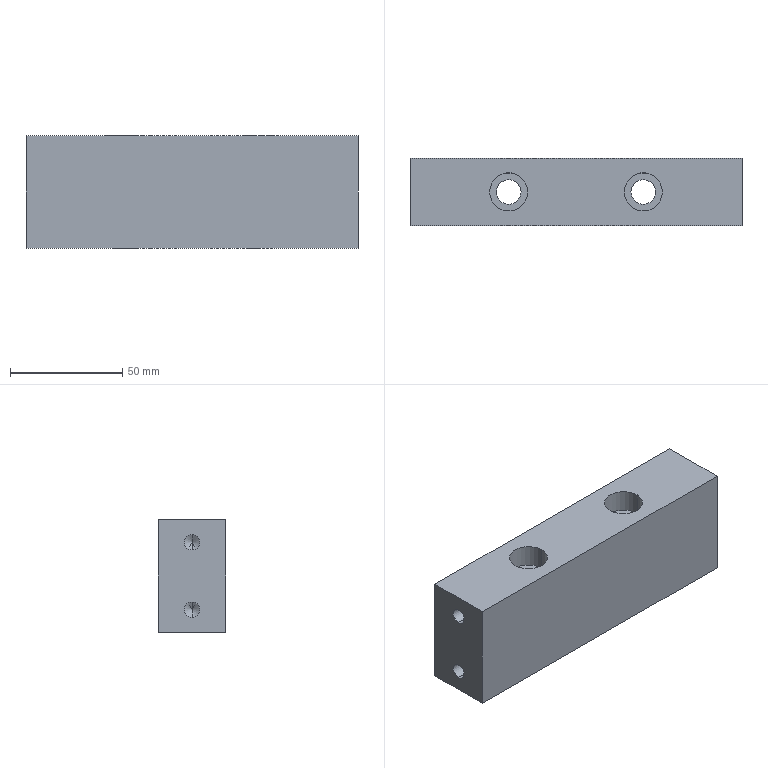Component | SolidWorks | GuideMechanism-1_GuideSeatFixingPlate-1 | 1 solid | 32 faces | box 148 x 30 x 50 mm | volume 207289 mm3 | cylinder 16 | cone 8 | plane 8 | commonest cylinder face diameters 6.8 x8 17 x4 11 x4
build123d program:
from build123d import *

# Parameters (mm, degrees)
SKETCH1_W                                        = 148
SKETCH1_H                                        = 30
BOSS_EXTRUDE1_DEPTH                              = 50
HOLE_SIZE_ACCORDING_TO_TYPE_1_OF_HEX_D           = 11
HOLE_SIZE_ACCORDING_TO_TYPE_1_OF_HEX_CBORE_D     = 17
HOLE_SIZE_ACCORDING_TO_TYPE_1_OF_HEX_CBORE_DEPTH = 10
M8_TAPPED_HOLE1_AT_2_COUNT                       = 2
M8_TAPPED_HOLE1_AT_2_PITCH                       = 30


with BuildPart() as part:
    # Sketch1 → Boss-Extrude1 (new body)
    with BuildSketch(Plane.XY):
        Rectangle(SKETCH1_W, SKETCH1_H)
    extrude(amount=BOSS_EXTRUDE1_DEPTH)

    # Hole Size _ according to_ Type 1 of Hex (through all)
    with Locations(Plane.XY.offset(50)):
        with Locations((-30, 0), (30, 0)):
            CounterBoreHole(HOLE_SIZE_ACCORDING_TO_TYPE_1_OF_HEX_D / 2, HOLE_SIZE_ACCORDING_TO_TYPE_1_OF_HEX_CBORE_D / 2, HOLE_SIZE_ACCORDING_TO_TYPE_1_OF_HEX_CBORE_DEPTH)

    # Sketch6 → M8 Tapped Hole1 (revolve, cut)
    with BuildSketch(Plane(origin=(74, 0, 40), x_dir=(0, 0, -1), z_dir=(0, 1, 0))):
        Polygon((0, 0), (0, 19.043), (3.4, 17), (3.4, 0), align=None)
    m8_tapped_hole1 = revolve(axis=Axis((80.35, 0, 40), (-1, 0, 0)), mode=Mode.SUBTRACT)

    # M8 Tapped Hole1 at 2: M8 Tapped Hole1 ×2
    with Locations(*[(0, 0, -i * M8_TAPPED_HOLE1_AT_2_PITCH) for i in range(1, M8_TAPPED_HOLE1_AT_2_COUNT)]):
        add(m8_tapped_hole1, mode=Mode.SUBTRACT)

    # Mirror1: M8 Tapped Hole1 across plane
    add(m8_tapped_hole1.mirror(Plane(origin=(0, 0, 0), x_dir=(0, 0, 1), z_dir=(1, 0, 0))), mode=Mode.SUBTRACT)

    # Mirror1 copy 1 sketch → Mirror1 copy 1 (revolve, cut)
    with BuildSketch(Plane(origin=(-74, 0, 10), x_dir=(0, 0, -1), z_dir=(0, 1, 0))):
        Polygon((0, 0), (0, -19.043), (3.4, -17), (3.4, 0), align=None)
    revolve(axis=Axis((-80.35, 0, 10), (-1, 0, 0)), mode=Mode.SUBTRACT)


solid = part.part

# Placed as in the assembly
solid = solid.moved(Location((-439.272, -538.766, 1161.5), (0, 0, 0)))
STEP:
#1=CARTESIAN_POINT('',(-19.538,-21.211,47.169));
#2=VERTEX_POINT('',#1);
#3=CARTESIAN_POINT('',(-19.538,-21.211,47.437));
#4=VERTEX_POINT('',#3);
#5=CARTESIAN_POINT('',(-19.538,-21.211,47.303));
#6=DIRECTION('',(-1.,0.,0.));
#7=DIRECTION('',(0.,0.,1.));
#8=AXIS2_PLACEMENT_3D('',#5,#6,#7);
#9=CIRCLE('',#8,0.1339);
#10=EDGE_CURVE('',#2,#4,#9,.T.);
#11=ORIENTED_EDGE('',*,*,#10,.F.);
#12=CARTESIAN_POINT('',(-20.208,-21.211,47.169));
#13=VERTEX_POINT('',#12);
#14=CARTESIAN_POINT('',(-20.208,-21.211,47.169));
#15=DIRECTION('',(-1.,0.,0.));
#16=VECTOR('',#15,39.37);
#17=LINE('',#14,#16);
#18=EDGE_CURVE('',#2,#13,#17,.T.);
#19=ORIENTED_EDGE('',*,*,#18,.T.);
#20=CARTESIAN_POINT('',(-20.208,-21.211,47.437));
#21=VERTEX_POINT('',#20);
#22=CARTESIAN_POINT('',(-20.208,-21.211,47.303));
#23=DIRECTION('',(-1.,0.,0.));
#24=DIRECTION('',(0.,0.,1.));
#25=AXIS2_PLACEMENT_3D('',#22,#23,#24);
#26=CIRCLE('',#25,0.1339);
#27=EDGE_CURVE('',#13,#21,#26,.T.);
#28=ORIENTED_EDGE('',*,*,#27,.T.);
#29=CARTESIAN_POINT('',(-20.208,-21.211,47.437));
#30=DIRECTION('',(-1.,0.,0.));
#31=VECTOR('',#30,39.37);
#32=LINE('',#29,#31);
#33=EDGE_CURVE('',#4,#21,#32,.T.);
#34=ORIENTED_EDGE('',*,*,#33,.F.);
#35=EDGE_LOOP('',(#11,#19,#28,#34));
#36=FACE_OUTER_BOUND('',#35,.T.);
#37=CARTESIAN_POINT('',(-20.208,-21.211,47.303));
#38=DIRECTION('',(-1.,0.,0.));
#39=DIRECTION('',(0.,0.,1.));
#40=AXIS2_PLACEMENT_3D('',#37,#38,#39);
#41=CYLINDRICAL_SURFACE('',#40,0.1339);
#42=ADVANCED_FACE('',(#36),#41,.F.);
#43=CARTESIAN_POINT('',(-19.458,-21.211,47.303));
#44=VERTEX_POINT('',#43);
#45=CARTESIAN_POINT('',(-19.538,-21.211,47.437));
#46=DIRECTION('',(-0.515,0.,0.8572));
#47=VECTOR('',#46,39.37);
#48=LINE('',#45,#47);
#49=EDGE_CURVE('',#44,#4,#48,.T.);
#50=ORIENTED_EDGE('',*,*,#49,.F.);
#51=CARTESIAN_POINT('',(-19.538,-21.211,47.169));
#52=DIRECTION('',(-0.515,0.,-0.8572));
#53=VECTOR('',#52,39.37);
#54=LINE('',#51,#53);
#55=EDGE_CURVE('',#44,#2,#54,.T.);
#56=ORIENTED_EDGE('',*,*,#55,.T.);
#57=ORIENTED_EDGE('',*,*,#10,.T.);
#58=EDGE_LOOP('',(#50,#56,#57));
#59=FACE_OUTER_BOUND('',#58,.T.);
#60=CARTESIAN_POINT('',(-19.538,-21.211,47.303));
#61=DIRECTION('',(-1.,0.,0.));
#62=DIRECTION('',(0.,0.,1.));
#63=AXIS2_PLACEMENT_3D('',#60,#61,#62);
#64=CONICAL_SURFACE('',#63,0.1339,1.03);
#65=ADVANCED_FACE('',(#59),#64,.F.);
#66=CARTESIAN_POINT('',(-19.538,-21.211,45.988));
#67=VERTEX_POINT('',#66);
#68=CARTESIAN_POINT('',(-19.538,-21.211,46.256));
#69=VERTEX_POINT('',#68);
#70=CARTESIAN_POINT('',(-19.538,-21.211,46.122));
#71=DIRECTION('',(-1.,0.,0.));
#72=DIRECTION('',(0.,0.,1.));
#73=AXIS2_PLACEMENT_3D('',#70,#71,#72);
#74=CIRCLE('',#73,0.1339);
#75=EDGE_CURVE('',#67,#69,#74,.T.);
#76=ORIENTED_EDGE('',*,*,#75,.F.);
#77=CARTESIAN_POINT('',(-20.208,-21.211,45.988));
#78=VERTEX_POINT('',#77);
#79=CARTESIAN_POINT('',(-20.208,-21.211,45.988));
#80=DIRECTION('',(-1.,0.,0.));
#81=VECTOR('',#80,39.37);
#82=LINE('',#79,#81);
#83=EDGE_CURVE('',#67,#78,#82,.T.);
#84=ORIENTED_EDGE('',*,*,#83,.T.);
#85=CARTESIAN_POINT('',(-20.208,-21.211,46.256));
#86=VERTEX_POINT('',#85);
#87=CARTESIAN_POINT('',(-20.208,-21.211,46.122));
#88=DIRECTION('',(-1.,0.,0.));
#89=DIRECTION('',(0.,0.,1.));
#90=AXIS2_PLACEMENT_3D('',#87,#88,#89);
#91=CIRCLE('',#90,0.1339);
#92=EDGE_CURVE('',#78,#86,#91,.T.);
#93=ORIENTED_EDGE('',*,*,#92,.T.);
#94=CARTESIAN_POINT('',(-20.208,-21.211,46.256));
#95=DIRECTION('',(-1.,0.,0.));
#96=VECTOR('',#95,39.37);
#97=LINE('',#94,#96);
#98=EDGE_CURVE('',#69,#86,#97,.T.);
#99=ORIENTED_EDGE('',*,*,#98,.F.);
#100=EDGE_LOOP('',(#76,#84,#93,#99));
#101=FACE_OUTER_BOUND('',#100,.T.);
#102=CARTESIAN_POINT('',(-20.208,-21.211,46.122));
#103=DIRECTION('',(-1.,0.,0.));
#104=DIRECTION('',(0.,0.,1.));
#105=AXIS2_PLACEMENT_3D('',#102,#103,#104);
#106=CYLINDRICAL_SURFACE('',#105,0.1339);
#107=ADVANCED_FACE('',(#101),#106,.F.);
#108=CARTESIAN_POINT('',(-19.458,-21.211,46.122));
#109=VERTEX_POINT('',#108);
#110=CARTESIAN_POINT('',(-19.538,-21.211,46.256));
#111=DIRECTION('',(-0.515,0.,0.8572));
#112=VECTOR('',#111,39.37);
#113=LINE('',#110,#112);
#114=EDGE_CURVE('',#109,#69,#113,.T.);
#115=ORIENTED_EDGE('',*,*,#114,.F.);
#116=CARTESIAN_POINT('',(-19.538,-21.211,45.988));
#117=DIRECTION('',(-0.515,0.,-0.8572));
#118=VECTOR('',#117,39.37);
#119=LINE('',#116,#118);
#120=EDGE_CURVE('',#109,#67,#119,.T.);
#121=ORIENTED_EDGE('',*,*,#120,.T.);
#122=ORIENTED_EDGE('',*,*,#75,.T.);
#123=EDGE_LOOP('',(#115,#121,#122));
#124=FACE_OUTER_BOUND('',#123,.T.);
#125=CARTESIAN_POINT('',(-19.538,-21.211,46.122));
#126=DIRECTION('',(-1.,0.,0.));
#127=DIRECTION('',(0.,0.,1.));
#128=AXIS2_PLACEMENT_3D('',#125,#126,#127);
#129=CONICAL_SURFACE('',#128,0.1339,1.03);
#130=ADVANCED_FACE('',(#124),#129,.F.);
#131=CARTESIAN_POINT('',(-15.05,-21.211,47.437));
#132=VERTEX_POINT('',#131);
#133=CARTESIAN_POINT('',(-15.05,-21.211,47.169));
#134=VERTEX_POINT('',#133);
#135=CARTESIAN_POINT('',(-15.05,-21.211,47.303));
#136=DIRECTION('',(1.,0.,0.));
#137=DIRECTION('',(0.,0.,-1.));
#138=AXIS2_PLACEMENT_3D('',#135,#136,#137);
#139=CIRCLE('',#138,0.1339);
#140=EDGE_CURVE('',#132,#134,#139,.T.);
#141=ORIENTED_EDGE('',*,*,#140,.F.);
#142=CARTESIAN_POINT('',(-14.381,-21.211,47.437));
#143=VERTEX_POINT('',#142);
#144=CARTESIAN_POINT('',(-14.381,-21.211,47.437));
#145=DIRECTION('',(1.,0.,0.));
#146=VECTOR('',#145,39.37);
#147=LINE('',#144,#146);
#148=EDGE_CURVE('',#132,#143,#147,.T.);
#149=ORIENTED_EDGE('',*,*,#148,.T.);
#150=CARTESIAN_POINT('',(-14.381,-21.211,47.169));
#151=VERTEX_POINT('',#150);
#152=CARTESIAN_POINT('',(-14.381,-21.211,47.303));
#153=DIRECTION('',(1.,0.,0.));
#154=DIRECTION('',(0.,0.,-1.));
#155=AXIS2_PLACEMENT_3D('',#152,#153,#154);
#156=CIRCLE('',#155,0.1339);
#157=EDGE_CURVE('',#143,#151,#156,.T.);
#158=ORIENTED_EDGE('',*,*,#157,.T.);
#159=CARTESIAN_POINT('',(-14.381,-21.211,47.169));
#160=DIRECTION('',(1.,0.,0.));
#161=VECTOR('',#160,39.37);
#162=LINE('',#159,#161);
#163=EDGE_CURVE('',#134,#151,#162,.T.);
#164=ORIENTED_EDGE('',*,*,#163,.F.);
#165=EDGE_LOOP('',(#141,#149,#158,#164));
#166=FACE_OUTER_BOUND('',#165,.T.);
#167=CARTESIAN_POINT('',(-14.381,-21.211,47.303));
#168=DIRECTION('',(1.,0.,0.));
#169=DIRECTION('',(0.,0.,-1.));
#170=AXIS2_PLACEMENT_3D('',#167,#168,#169);
#171=CYLINDRICAL_SURFACE('',#170,0.1339);
#172=ADVANCED_FACE('',(#166),#171,.F.);
#173=CARTESIAN_POINT('',(-15.131,-21.211,47.303));
#174=VERTEX_POINT('',#173);
#175=CARTESIAN_POINT('',(-15.05,-21.211,47.169));
#176=DIRECTION('',(0.515,0.,-0.8572));
#177=VECTOR('',#176,39.37);
#178=LINE('',#175,#177);
#179=EDGE_CURVE('',#174,#134,#178,.T.);
#180=ORIENTED_EDGE('',*,*,#179,.F.);
#181=CARTESIAN_POINT('',(-15.05,-21.211,47.437));
#182=DIRECTION('',(0.515,0.,0.8572));
#183=VECTOR('',#182,39.37);
#184=LINE('',#181,#183);
#185=EDGE_CURVE('',#174,#132,#184,.T.);
#186=ORIENTED_EDGE('',*,*,#185,.T.);
#187=ORIENTED_EDGE('',*,*,#140,.T.);
#188=EDGE_LOOP('',(#180,#186,#187));
#189=FACE_OUTER_BOUND('',#188,.T.);
#190=CARTESIAN_POINT('',(-15.05,-21.211,47.303));
#191=DIRECTION('',(1.,0.,0.));
#192=DIRECTION('',(0.,0.,-1.));
#193=AXIS2_PLACEMENT_3D('',#190,#191,#192);
#194=CONICAL_SURFACE('',#193,0.1339,1.03);
#195=ADVANCED_FACE('',(#189),#194,.F.);
#196=CARTESIAN_POINT('',(-15.05,-21.211,46.256));
#197=VERTEX_POINT('',#196);
#198=CARTESIAN_POINT('',(-15.05,-21.211,45.988));
#199=VERTEX_POINT('',#198);
#200=CARTESIAN_POINT('',(-15.05,-21.211,46.122));
#201=DIRECTION('',(1.,0.,0.));
#202=DIRECTION('',(0.,0.,-1.));
#203=AXIS2_PLACEMENT_3D('',#200,#201,#202);
#204=CIRCLE('',#203,0.1339);
#205=EDGE_CURVE('',#197,#199,#204,.T.);
#206=ORIENTED_EDGE('',*,*,#205,.F.);
#207=CARTESIAN_POINT('',(-14.381,-21.211,46.256));
#208=VERTEX_POINT('',#207);
#209=CARTESIAN_POINT('',(-14.381,-21.211,46.256));
#210=DIRECTION('',(1.,0.,0.));
#211=VECTOR('',#210,39.37);
#212=LINE('',#209,#211);
#213=EDGE_CURVE('',#197,#208,#212,.T.);
#214=ORIENTED_EDGE('',*,*,#213,.T.);
#215=CARTESIAN_POINT('',(-14.381,-21.211,45.988));
#216=VERTEX_POINT('',#215);
#217=CARTESIAN_POINT('',(-14.381,-21.211,46.122));
#218=DIRECTION('',(1.,0.,0.));
#219=DIRECTION('',(0.,0.,-1.));
#220=AXIS2_PLACEMENT_3D('',#217,#218,#219);
#221=CIRCLE('',#220,0.1339);
#222=EDGE_CURVE('',#208,#216,#221,.T.);
#223=ORIENTED_EDGE('',*,*,#222,.T.);
#224=CARTESIAN_POINT('',(-14.381,-21.211,45.988));
#225=DIRECTION('',(1.,0.,0.));
#226=VECTOR('',#225,39.37);
#227=LINE('',#224,#226);
#228=EDGE_CURVE('',#199,#216,#227,.T.);
#229=ORIENTED_EDGE('',*,*,#228,.F.);
#230=EDGE_LOOP('',(#206,#214,#223,#229));
#231=FACE_OUTER_BOUND('',#230,.T.);
#232=CARTESIAN_POINT('',(-14.381,-21.211,46.122));
#233=DIRECTION('',(1.,0.,0.));
#234=DIRECTION('',(0.,0.,-1.));
#235=AXIS2_PLACEMENT_3D('',#232,#233,#234);
#236=CYLINDRICAL_SURFACE('',#235,0.1339);
#237=ADVANCED_FACE('',(#231),#236,.F.);
#238=CARTESIAN_POINT('',(-15.131,-21.211,46.122));
#239=VERTEX_POINT('',#238);
#240=CARTESIAN_POINT('',(-15.05,-21.211,45.988));
#241=DIRECTION('',(0.515,0.,-0.8572));
#242=VECTOR('',#241,39.37);
#243=LINE('',#240,#242);
#244=EDGE_CURVE('',#239,#199,#243,.T.);
#245=ORIENTED_EDGE('',*,*,#244,.F.);
#246=CARTESIAN_POINT('',(-15.05,-21.211,46.256));
#247=DIRECTION('',(0.515,0.,0.8572));
#248=VECTOR('',#247,39.37);
#249=LINE('',#246,#248);
#250=EDGE_CURVE('',#239,#197,#249,.T.);
#251=ORIENTED_EDGE('',*,*,#250,.T.);
#252=ORIENTED_EDGE('',*,*,#205,.T.);
#253=EDGE_LOOP('',(#245,#251,#252));
#254=FACE_OUTER_BOUND('',#253,.T.);
#255=CARTESIAN_POINT('',(-15.05,-21.211,46.122));
#256=DIRECTION('',(1.,0.,0.));
#257=DIRECTION('',(0.,0.,-1.));
#258=AXIS2_PLACEMENT_3D('',#255,#256,#257);
#259=CONICAL_SURFACE('',#258,0.1339,1.03);
#260=ADVANCED_FACE('',(#254),#259,.F.);
#261=CARTESIAN_POINT('',(-18.81,-21.211,47.303));
#262=VERTEX_POINT('',#261);
#263=CARTESIAN_POINT('',(-18.141,-21.211,47.303));
#264=VERTEX_POINT('',#263);
#265=CARTESIAN_POINT('',(-18.475,-21.211,47.303));
#266=DIRECTION('',(0.,0.,1.));
#267=DIRECTION('',(1.,0.,0.));
#268=AXIS2_PLACEMENT_3D('',#265,#266,#267);
#269=CIRCLE('',#268,0.3346);
#270=EDGE_CURVE('',#262,#264,#269,.T.);
#271=ORIENTED_EDGE('',*,*,#270,.F.);
#272=CARTESIAN_POINT('',(-18.81,-21.211,47.697));
#273=VERTEX_POINT('',#272);
#274=CARTESIAN_POINT('',(-18.81,-21.211,47.697));
#275=DIRECTION('',(0.,0.,1.));
#276=VECTOR('',#275,39.37);
#277=LINE('',#274,#276);
#278=EDGE_CURVE('',#262,#273,#277,.T.);
#279=ORIENTED_EDGE('',*,*,#278,.T.);
#280=CARTESIAN_POINT('',(-18.141,-21.211,47.697));
#281=VERTEX_POINT('',#280);
#282=CARTESIAN_POINT('',(-18.475,-21.211,47.697));
#283=DIRECTION('',(0.,0.,1.));
#284=DIRECTION('',(1.,0.,0.));
#285=AXIS2_PLACEMENT_3D('',#282,#283,#284);
#286=CIRCLE('',#285,0.3346);
#287=EDGE_CURVE('',#273,#281,#286,.T.);
#288=ORIENTED_EDGE('',*,*,#287,.T.);
#289=CARTESIAN_POINT('',(-18.141,-21.211,47.697));
#290=DIRECTION('',(0.,0.,1.));
#291=VECTOR('',#290,39.37);
#292=LINE('',#289,#291);
#293=EDGE_CURVE('',#264,#281,#292,.T.);
#294=ORIENTED_EDGE('',*,*,#293,.F.);
#295=EDGE_LOOP('',(#271,#279,#288,#294));
#296=FACE_OUTER_BOUND('',#295,.T.);
#297=CARTESIAN_POINT('',(-18.475,-21.211,47.697));
#298=DIRECTION('',(0.,0.,1.));
#299=DIRECTION('',(1.,0.,0.));
#300=AXIS2_PLACEMENT_3D('',#297,#298,#299);
#301=CYLINDRICAL_SURFACE('',#300,0.3346);
#302=ADVANCED_FACE('',(#296),#301,.F.);
#303=CARTESIAN_POINT('',(-18.692,-21.211,45.728));
#304=VERTEX_POINT('',#303);
#305=CARTESIAN_POINT('',(-18.259,-21.211,45.728));
#306=VERTEX_POINT('',#305);
#307=CARTESIAN_POINT('',(-18.475,-21.211,45.728));
#308=DIRECTION('',(0.,0.,1.));
#309=DIRECTION('',(1.,0.,0.));
#310=AXIS2_PLACEMENT_3D('',#307,#308,#309);
#311=CIRCLE('',#310,0.2165);
#312=EDGE_CURVE('',#304,#306,#311,.T.);
#313=ORIENTED_EDGE('',*,*,#312,.F.);
#314=CARTESIAN_POINT('',(-18.692,-21.211,47.303));
#315=VERTEX_POINT('',#314);
#316=CARTESIAN_POINT('',(-18.692,-21.211,47.697));
#317=DIRECTION('',(0.,0.,1.));
#318=VECTOR('',#317,39.37);
#319=LINE('',#316,#318);
#320=EDGE_CURVE('',#304,#315,#319,.T.);
#321=ORIENTED_EDGE('',*,*,#320,.T.);
#322=CARTESIAN_POINT('',(-18.259,-21.211,47.303));
#323=VERTEX_POINT('',#322);
#324=CARTESIAN_POINT('',(-18.475,-21.211,47.303));
#325=DIRECTION('',(0.,0.,1.));
#326=DIRECTION('',(1.,0.,0.));
#327=AXIS2_PLACEMENT_3D('',#324,#325,#326);
#328=CIRCLE('',#327,0.2165);
#329=EDGE_CURVE('',#315,#323,#328,.T.);
#330=ORIENTED_EDGE('',*,*,#329,.T.);
#331=CARTESIAN_POINT('',(-18.259,-21.211,47.697));
#332=DIRECTION('',(0.,0.,1.));
#333=VECTOR('',#332,39.37);
#334=LINE('',#331,#333);
#335=EDGE_CURVE('',#306,#323,#334,.T.);
#336=ORIENTED_EDGE('',*,*,#335,.F.);
#337=EDGE_LOOP('',(#313,#321,#330,#336));
#338=FACE_OUTER_BOUND('',#337,.T.);
#339=CARTESIAN_POINT('',(-18.475,-21.211,47.697));
#340=DIRECTION('',(0.,0.,1.));
#341=DIRECTION('',(1.,0.,0.));
#342=AXIS2_PLACEMENT_3D('',#339,#340,#341);
#343=CYLINDRICAL_SURFACE('',#342,0.2165);
#344=ADVANCED_FACE('',(#338),#343,.F.);
#345=CARTESIAN_POINT('',(-16.448,-21.211,47.303));
#346=VERTEX_POINT('',#345);
#347=CARTESIAN_POINT('',(-15.778,-21.211,47.303));
#348=VERTEX_POINT('',#347);
#349=CARTESIAN_POINT('',(-16.113,-21.211,47.303));
#350=DIRECTION('',(0.,0.,1.));
#351=DIRECTION('',(1.,0.,0.));
#352=AXIS2_PLACEMENT_3D('',#349,#350,#351);
#353=CIRCLE('',#352,0.3346);
#354=EDGE_CURVE('',#346,#348,#353,.T.);
#355=ORIENTED_EDGE('',*,*,#354,.F.);
#356=CARTESIAN_POINT('',(-16.448,-21.211,47.697));
#357=VERTEX_POINT('',#356);
#358=CARTESIAN_POINT('',(-16.448,-21.211,47.697));
#359=DIRECTION('',(0.,0.,1.));
#360=VECTOR('',#359,39.37);
#361=LINE('',#358,#360);
#362=EDGE_CURVE('',#346,#357,#361,.T.);
#363=ORIENTED_EDGE('',*,*,#362,.T.);
#364=CARTESIAN_POINT('',(-15.778,-21.211,47.697));
#365=VERTEX_POINT('',#364);
#366=CARTESIAN_POINT('',(-16.113,-21.211,47.697));
#367=DIRECTION('',(0.,0.,1.));
#368=DIRECTION('',(1.,0.,0.));
#369=AXIS2_PLACEMENT_3D('',#366,#367,#368);
#370=CIRCLE('',#369,0.3346);
#371=EDGE_CURVE('',#357,#365,#370,.T.);
#372=ORIENTED_EDGE('',*,*,#371,.T.);
#373=CARTESIAN_POINT('',(-15.778,-21.211,47.697));
#374=DIRECTION('',(0.,0.,1.));
#375=VECTOR('',#374,39.37);
#376=LINE('',#373,#375);
#377=EDGE_CURVE('',#348,#365,#376,.T.);
#378=ORIENTED_EDGE('',*,*,#377,.F.);
#379=EDGE_LOOP('',(#355,#363,#372,#378));
#380=FACE_OUTER_BOUND('',#379,.T.);
#381=CARTESIAN_POINT('',(-16.113,-21.211,47.697));
#382=DIRECTION('',(0.,0.,1.));
#383=DIRECTION('',(1.,0.,0.));
#384=AXIS2_PLACEMENT_3D('',#381,#382,#383);
#385=CYLINDRICAL_SURFACE('',#384,0.3346);
#386=ADVANCED_FACE('',(#380),#385,.F.);
#387=CARTESIAN_POINT('',(-16.33,-21.211,45.728));
#388=VERTEX_POINT('',#387);
#389=CARTESIAN_POINT('',(-15.897,-21.211,45.728));
#390=VERTEX_POINT('',#389);
#391=CARTESIAN_POINT('',(-16.113,-21.211,45.728));
#392=DIRECTION('',(0.,0.,1.));
#393=DIRECTION('',(1.,0.,0.));
#394=AXIS2_PLACEMENT_3D('',#391,#392,#393);
#395=CIRCLE('',#394,0.2165);
#396=EDGE_CURVE('',#388,#390,#395,.T.);
#397=ORIENTED_EDGE('',*,*,#396,.F.);
#398=CARTESIAN_POINT('',(-16.33,-21.211,47.303));
#399=VERTEX_POINT('',#398);
#400=CARTESIAN_POINT('',(-16.33,-21.211,47.697));
#401=DIRECTION('',(0.,0.,1.));
#402=VECTOR('',#401,39.37);
#403=LINE('',#400,#402);
#404=EDGE_CURVE('',#388,#399,#403,.T.);
#405=ORIENTED_EDGE('',*,*,#404,.T.);
#406=CARTESIAN_POINT('',(-15.897,-21.211,47.303));
#407=VERTEX_POINT('',#406);
#408=CARTESIAN_POINT('',(-16.113,-21.211,47.303));
#409=DIRECTION('',(0.,0.,1.));
#410=DIRECTION('',(1.,0.,0.));
#411=AXIS2_PLACEMENT_3D('',#408,#409,#410);
#412=CIRCLE('',#411,0.2165);
#413=EDGE_CURVE('',#399,#407,#412,.T.);
#414=ORIENTED_EDGE('',*,*,#413,.T.);
#415=CARTESIAN_POINT('',(-15.897,-21.211,47.697));
#416=DIRECTION('',(0.,0.,1.));
#417=VECTOR('',#416,39.37);
#418=LINE('',#415,#417);
#419=EDGE_CURVE('',#390,#407,#418,.T.);
#420=ORIENTED_EDGE('',*,*,#419,.F.);
#421=EDGE_LOOP('',(#397,#405,#414,#420));
#422=FACE_OUTER_BOUND('',#421,.T.);
#423=CARTESIAN_POINT('',(-16.113,-21.211,47.697));
#424=DIRECTION('',(0.,0.,1.));
#425=DIRECTION('',(1.,0.,0.));
#426=AXIS2_PLACEMENT_3D('',#423,#424,#425);
#427=CYLINDRICAL_SURFACE('',#426,0.2165);
#428=ADVANCED_FACE('',(#422),#427,.F.);
#429=CARTESIAN_POINT('',(-20.208,-21.211,47.303));
#430=DIRECTION('',(-1.,0.,0.));
#431=DIRECTION('',(0.,0.,1.));
#432=AXIS2_PLACEMENT_3D('',#429,#430,#431);
#433=CIRCLE('',#432,0.1339);
#434=EDGE_CURVE('',#21,#13,#433,.T.);
#435=ORIENTED_EDGE('',*,*,#434,.F.);
#436=ORIENTED_EDGE('',*,*,#27,.F.);
#437=EDGE_LOOP('',(#435,#436));
#438=FACE_BOUND('',#437,.T.);
#439=CARTESIAN_POINT('',(-20.208,-21.211,46.122));
#440=DIRECTION('',(-1.,0.,0.));
#441=DIRECTION('',(0.,0.,1.));
#442=AXIS2_PLACEMENT_3D('',#439,#440,#441);
#443=CIRCLE('',#442,0.1339);
#444=EDGE_CURVE('',#86,#78,#443,.T.);
#445=ORIENTED_EDGE('',*,*,#444,.F.);
#446=ORIENTED_EDGE('',*,*,#92,.F.);
#447=EDGE_LOOP('',(#445,#446));
#448=FACE_BOUND('',#447,.T.);
#449=CARTESIAN_POINT('',(-20.208,-20.621,45.728));
#450=VERTEX_POINT('',#449);
#451=CARTESIAN_POINT('',(-20.208,-21.802,45.728));
#452=VERTEX_POINT('',#451);
#453=CARTESIAN_POINT('',(-20.208,-21.802,45.728));
#454=DIRECTION('',(0.,-1.,0.));
#455=VECTOR('',#454,39.37);
#456=LINE('',#453,#455);
#457=EDGE_CURVE('',#450,#452,#456,.T.);
#458=ORIENTED_EDGE('',*,*,#457,.T.);
#459=CARTESIAN_POINT('',(-20.208,-21.802,47.697));
#460=VERTEX_POINT('',#459);
#461=CARTESIAN_POINT('',(-20.208,-21.802,47.697));
#462=DIRECTION('',(0.,0.,-1.));
#463=VECTOR('',#462,39.37);
#464=LINE('',#461,#463);
#465=EDGE_CURVE('',#460,#452,#464,.T.);
#466=ORIENTED_EDGE('',*,*,#465,.F.);
#467=CARTESIAN_POINT('',(-20.208,-20.621,47.697));
#468=VERTEX_POINT('',#467);
#469=CARTESIAN_POINT('',(-20.208,-21.802,47.697));
#470=DIRECTION('',(0.,-1.,0.));
#471=VECTOR('',#470,39.37);
#472=LINE('',#469,#471);
#473=EDGE_CURVE('',#468,#460,#472,.T.);
#474=ORIENTED_EDGE('',*,*,#473,.F.);
#475=CARTESIAN_POINT('',(-20.208,-20.621,47.697));
#476=DIRECTION('',(0.,0.,-1.));
#477=VECTOR('',#476,39.37);
#478=LINE('',#475,#477);
#479=EDGE_CURVE('',#468,#450,#478,.T.);
#480=ORIENTED_EDGE('',*,*,#479,.T.);
#481=EDGE_LOOP('',(#458,#466,#474,#480));
#482=FACE_OUTER_BOUND('',#481,.T.);
#483=CARTESIAN_POINT('',(-20.208,-21.802,47.697));
#484=DIRECTION('',(1.,0.,0.));
#485=DIRECTION('',(0.,0.,-1.));
#486=AXIS2_PLACEMENT_3D('',#483,#484,#485);
#487=PLANE('',#486);
#488=ADVANCED_FACE('',(#438,#448,#482),#487,.F.);
#489=CARTESIAN_POINT('',(-14.381,-21.802,45.728));
#490=VERTEX_POINT('',#489);
#491=CARTESIAN_POINT('',(-14.381,-21.802,45.728));
#492=DIRECTION('',(1.,0.,0.));
#493=VECTOR('',#492,39.37);
#494=LINE('',#491,#493);
#495=EDGE_CURVE('',#452,#490,#494,.T.);
#496=ORIENTED_EDGE('',*,*,#495,.T.);
#497=CARTESIAN_POINT('',(-14.381,-21.802,47.697));
#498=VERTEX_POINT('',#497);
#499=CARTESIAN_POINT('',(-14.381,-21.802,47.697));
#500=DIRECTION('',(0.,0.,-1.));
#501=VECTOR('',#500,39.37);
#502=LINE('',#499,#501);
#503=EDGE_CURVE('',#498,#490,#502,.T.);
#504=ORIENTED_EDGE('',*,*,#503,.F.);
#505=CARTESIAN_POINT('',(-14.381,-21.802,47.697));
#506=DIRECTION('',(1.,0.,0.));
#507=VECTOR('',#506,39.37);
#508=LINE('',#505,#507);
#509=EDGE_CURVE('',#460,#498,#508,.T.);
#510=ORIENTED_EDGE('',*,*,#509,.F.);
#511=ORIENTED_EDGE('',*,*,#465,.T.);
#512=EDGE_LOOP('',(#496,#504,#510,#511));
#513=FACE_OUTER_BOUND('',#512,.T.);
#514=CARTESIAN_POINT('',(-14.381,-21.802,47.697));
#515=DIRECTION('',(-0.,1.,0.));
#516=DIRECTION('',(-1.,-0.,0.));
#517=AXIS2_PLACEMENT_3D('',#514,#515,#516);
#518=PLANE('',#517);
#519=ADVANCED_FACE('',(#513),#518,.F.);
#520=CARTESIAN_POINT('',(-14.381,-21.211,47.303));
#521=DIRECTION('',(1.,0.,0.));
#522=DIRECTION('',(0.,0.,-1.));
#523=AXIS2_PLACEMENT_3D('',#520,#521,#522);
#524=CIRCLE('',#523,0.1339);
#525=EDGE_CURVE('',#151,#143,#524,.T.);
#526=ORIENTED_EDGE('',*,*,#525,.F.);
#527=ORIENTED_EDGE('',*,*,#157,.F.);
#528=EDGE_LOOP('',(#526,#527));
#529=FACE_BOUND('',#528,.T.);
#530=CARTESIAN_POINT('',(-14.381,-21.211,46.122));
#531=DIRECTION('',(1.,0.,0.));
#532=DIRECTION('',(0.,0.,-1.));
#533=AXIS2_PLACEMENT_3D('',#530,#531,#532);
#534=CIRCLE('',#533,0.1339);
#535=EDGE_CURVE('',#216,#208,#534,.T.);
#536=ORIENTED_EDGE('',*,*,#535,.F.);
#537=ORIENTED_EDGE('',*,*,#222,.F.);
#538=EDGE_LOOP('',(#536,#537));
#539=FACE_BOUND('',#538,.T.);
#540=CARTESIAN_POINT('',(-14.381,-20.621,45.728));
#541=VERTEX_POINT('',#540);
#542=CARTESIAN_POINT('',(-14.381,-21.802,45.728));
#543=DIRECTION('',(0.,1.,0.));
#544=VECTOR('',#543,39.37);
#545=LINE('',#542,#544);
#546=EDGE_CURVE('',#490,#541,#545,.T.);
#547=ORIENTED_EDGE('',*,*,#546,.T.);
#548=CARTESIAN_POINT('',(-14.381,-20.621,47.697));
#549=VERTEX_POINT('',#548);
#550=CARTESIAN_POINT('',(-14.381,-20.621,47.697));
#551=DIRECTION('',(0.,0.,-1.));
#552=VECTOR('',#551,39.37);
#553=LINE('',#550,#552);
#554=EDGE_CURVE('',#549,#541,#553,.T.);
#555=ORIENTED_EDGE('',*,*,#554,.F.);
#556=CARTESIAN_POINT('',(-14.381,-21.802,47.697));
#557=DIRECTION('',(0.,1.,0.));
#558=VECTOR('',#557,39.37);
#559=LINE('',#556,#558);
#560=EDGE_CURVE('',#498,#549,#559,.T.);
#561=ORIENTED_EDGE('',*,*,#560,.F.);
#562=ORIENTED_EDGE('',*,*,#503,.T.);
#563=EDGE_LOOP('',(#547,#555,#561,#562));
#564=FACE_OUTER_BOUND('',#563,.T.);
#565=CARTESIAN_POINT('',(-14.381,-21.802,47.697));
#566=DIRECTION('',(-1.,0.,0.));
#567=DIRECTION('',(0.,0.,1.));
#568=AXIS2_PLACEMENT_3D('',#565,#566,#567);
#569=PLANE('',#568);
#570=ADVANCED_FACE('',(#529,#539,#564),#569,.F.);
#571=CARTESIAN_POINT('',(-14.381,-20.621,45.728));
#572=DIRECTION('',(-1.,-0.,0.));
#573=VECTOR('',#572,39.37);
#574=LINE('',#571,#573);
#575=EDGE_CURVE('',#541,#450,#574,.T.);
#576=ORIENTED_EDGE('',*,*,#575,.T.);
#577=ORIENTED_EDGE('',*,*,#479,.F.);
#578=CARTESIAN_POINT('',(-14.381,-20.621,47.697));
#579=DIRECTION('',(-1.,-0.,0.));
#580=VECTOR('',#579,39.37);
#581=LINE('',#578,#580);
#582=EDGE_CURVE('',#549,#468,#581,.T.);
#583=ORIENTED_EDGE('',*,*,#582,.F.);
#584=ORIENTED_EDGE('',*,*,#554,.T.);
#585=EDGE_LOOP('',(#576,#577,#583,#584));
#586=FACE_OUTER_BOUND('',#585,.T.);
#587=CARTESIAN_POINT('',(-14.381,-20.621,47.697));
#588=DIRECTION('',(0.,-1.,0.));
#589=DIRECTION('',(1.,0.,0.));
#590=AXIS2_PLACEMENT_3D('',#587,#588,#589);
#591=PLANE('',#590);
#592=ADVANCED_FACE('',(#586),#591,.F.);
#593=CARTESIAN_POINT('',(-18.475,-21.211,47.697));
#594=DIRECTION('',(0.,0.,1.));
#595=DIRECTION('',(1.,0.,0.));
#596=AXIS2_PLACEMENT_3D('',#593,#594,#595);
#597=CIRCLE('',#596,0.3346);
#598=EDGE_CURVE('',#281,#273,#597,.T.);
#599=ORIENTED_EDGE('',*,*,#598,.F.);
#600=ORIENTED_EDGE('',*,*,#287,.F.);
#601=EDGE_LOOP('',(#599,#600));
#602=FACE_BOUND('',#601,.T.);
#603=CARTESIAN_POINT('',(-16.113,-21.211,47.697));
#604=DIRECTION('',(0.,0.,1.));
#605=DIRECTION('',(1.,0.,0.));
#606=AXIS2_PLACEMENT_3D('',#603,#604,#605);
#607=CIRCLE('',#606,0.3346);
#608=EDGE_CURVE('',#365,#357,#607,.T.);
#609=ORIENTED_EDGE('',*,*,#608,.F.);
#610=ORIENTED_EDGE('',*,*,#371,.F.);
#611=EDGE_LOOP('',(#609,#610));
#612=FACE_BOUND('',#611,.T.);
#613=ORIENTED_EDGE('',*,*,#473,.T.);
#614=ORIENTED_EDGE('',*,*,#509,.T.);
#615=ORIENTED_EDGE('',*,*,#560,.T.);
#616=ORIENTED_EDGE('',*,*,#582,.T.);
#617=EDGE_LOOP('',(#613,#614,#615,#616));
#618=FACE_OUTER_BOUND('',#617,.T.);
#619=CARTESIAN_POINT('',(-17.294,-21.211,47.697));
#620=DIRECTION('',(0.,0.,1.));
#621=DIRECTION('',(1.,0.,0.));
#622=AXIS2_PLACEMENT_3D('',#619,#620,#621);
#623=PLANE('',#622);
#624=ADVANCED_FACE('',(#602,#612,#618),#623,.T.);
#625=CARTESIAN_POINT('',(-18.475,-21.211,45.728));
#626=DIRECTION('',(0.,0.,1.));
#627=DIRECTION('',(1.,0.,0.));
#628=AXIS2_PLACEMENT_3D('',#625,#626,#627);
#629=CIRCLE('',#628,0.2165);
#630=EDGE_CURVE('',#306,#304,#629,.T.);
#631=ORIENTED_EDGE('',*,*,#630,.T.);
#632=ORIENTED_EDGE('',*,*,#312,.T.);
#633=EDGE_LOOP('',(#631,#632));
#634=FACE_BOUND('',#633,.T.);
#635=CARTESIAN_POINT('',(-16.113,-21.211,45.728));
#636=DIRECTION('',(0.,0.,1.));
#637=DIRECTION('',(1.,0.,0.));
#638=AXIS2_PLACEMENT_3D('',#635,#636,#637);
#639=CIRCLE('',#638,0.2165);
#640=EDGE_CURVE('',#390,#388,#639,.T.);
#641=ORIENTED_EDGE('',*,*,#640,.T.);
#642=ORIENTED_EDGE('',*,*,#396,.T.);
#643=EDGE_LOOP('',(#641,#642));
#644=FACE_BOUND('',#643,.T.);
#645=ORIENTED_EDGE('',*,*,#457,.F.);
#646=ORIENTED_EDGE('',*,*,#575,.F.);
#647=ORIENTED_EDGE('',*,*,#546,.F.);
#648=ORIENTED_EDGE('',*,*,#495,.F.);
#649=EDGE_LOOP('',(#645,#646,#647,#648));
#650=FACE_OUTER_BOUND('',#649,.T.);
#651=CARTESIAN_POINT('',(-17.294,-21.211,45.728));
#652=DIRECTION('',(0.,0.,1.));
#653=DIRECTION('',(1.,0.,0.));
#654=AXIS2_PLACEMENT_3D('',#651,#652,#653);
#655=PLANE('',#654);
#656=ADVANCED_FACE('',(#634,#644,#650),#655,.F.);
#657=ORIENTED_EDGE('',*,*,#404,.F.);
#658=ORIENTED_EDGE('',*,*,#640,.F.);
#659=ORIENTED_EDGE('',*,*,#419,.T.);
#660=CARTESIAN_POINT('',(-16.113,-21.211,47.303));
#661=DIRECTION('',(0.,0.,1.));
#662=DIRECTION('',(1.,0.,0.));
#663=AXIS2_PLACEMENT_3D('',#660,#661,#662);
#664=CIRCLE('',#663,0.2165);
#665=EDGE_CURVE('',#407,#399,#664,.T.);
#666=ORIENTED_EDGE('',*,*,#665,.T.);
#667=EDGE_LOOP('',(#657,#658,#659,#666));
#668=FACE_OUTER_BOUND('',#667,.T.);
#669=CARTESIAN_POINT('',(-16.113,-21.211,47.697));
#670=DIRECTION('',(0.,0.,1.));
#671=DIRECTION('',(1.,0.,0.));
#672=AXIS2_PLACEMENT_3D('',#669,#670,#671);
#673=CYLINDRICAL_SURFACE('',#672,0.2165);
#674=ADVANCED_FACE('',(#668),#673,.F.);
#675=ORIENTED_EDGE('',*,*,#665,.F.);
#676=ORIENTED_EDGE('',*,*,#413,.F.);
#677=EDGE_LOOP('',(#675,#676));
#678=FACE_BOUND('',#677,.T.);
#679=CARTESIAN_POINT('',(-16.113,-21.211,47.303));
#680=DIRECTION('',(0.,0.,1.));
#681=DIRECTION('',(1.,0.,0.));
#682=AXIS2_PLACEMENT_3D('',#679,#680,#681);
#683=CIRCLE('',#682,0.3346);
#684=EDGE_CURVE('',#348,#346,#683,.T.);
#685=ORIENTED_EDGE('',*,*,#684,.T.);
#686=ORIENTED_EDGE('',*,*,#354,.T.);
#687=EDGE_LOOP('',(#685,#686));
#688=FACE_OUTER_BOUND('',#687,.T.);
#689=CARTESIAN_POINT('',(-15.897,-21.211,47.303));
#690=DIRECTION('',(0.,0.,-1.));
#691=DIRECTION('',(-1.,0.,0.));
#692=AXIS2_PLACEMENT_3D('',#689,#690,#691);
#693=PLANE('',#692);
#694=ADVANCED_FACE('',(#678,#688),#693,.F.);
#695=ORIENTED_EDGE('',*,*,#362,.F.);
#696=ORIENTED_EDGE('',*,*,#684,.F.);
#697=ORIENTED_EDGE('',*,*,#377,.T.);
#698=ORIENTED_EDGE('',*,*,#608,.T.);
#699=EDGE_LOOP('',(#695,#696,#697,#698));
#700=FACE_OUTER_BOUND('',#699,.T.);
#701=CARTESIAN_POINT('',(-16.113,-21.211,47.697));
#702=DIRECTION('',(0.,0.,1.));
#703=DIRECTION('',(1.,0.,0.));
#704=AXIS2_PLACEMENT_3D('',#701,#702,#703);
#705=CYLINDRICAL_SURFACE('',#704,0.3346);
#706=ADVANCED_FACE('',(#700),#705,.F.);
#707=ORIENTED_EDGE('',*,*,#320,.F.);
#708=ORIENTED_EDGE('',*,*,#630,.F.);
#709=ORIENTED_EDGE('',*,*,#335,.T.);
#710=CARTESIAN_POINT('',(-18.475,-21.211,47.303));
#711=DIRECTION('',(0.,0.,1.));
#712=DIRECTION('',(1.,0.,0.));
#713=AXIS2_PLACEMENT_3D('',#710,#711,#712);
#714=CIRCLE('',#713,0.2165);
#715=EDGE_CURVE('',#323,#315,#714,.T.);
#716=ORIENTED_EDGE('',*,*,#715,.T.);
#717=EDGE_LOOP('',(#707,#708,#709,#716));
#718=FACE_OUTER_BOUND('',#717,.T.);
#719=CARTESIAN_POINT('',(-18.475,-21.211,47.697));
#720=DIRECTION('',(0.,0.,1.));
#721=DIRECTION('',(1.,0.,0.));
#722=AXIS2_PLACEMENT_3D('',#719,#720,#721);
#723=CYLINDRICAL_SURFACE('',#722,0.2165);
#724=ADVANCED_FACE('',(#718),#723,.F.);
#725=ORIENTED_EDGE('',*,*,#715,.F.);
#726=ORIENTED_EDGE('',*,*,#329,.F.);
#727=EDGE_LOOP('',(#725,#726));
#728=FACE_BOUND('',#727,.T.);
#729=CARTESIAN_POINT('',(-18.475,-21.211,47.303));
#730=DIRECTION('',(0.,0.,1.));
#731=DIRECTION('',(1.,0.,0.));
#732=AXIS2_PLACEMENT_3D('',#729,#730,#731);
#733=CIRCLE('',#732,0.3346);
#734=EDGE_CURVE('',#264,#262,#733,.T.);
#735=ORIENTED_EDGE('',*,*,#734,.T.);
#736=ORIENTED_EDGE('',*,*,#270,.T.);
#737=EDGE_LOOP('',(#735,#736));
#738=FACE_OUTER_BOUND('',#737,.T.);
#739=CARTESIAN_POINT('',(-18.259,-21.211,47.303));
#740=DIRECTION('',(0.,0.,-1.));
#741=DIRECTION('',(-1.,0.,0.));
#742=AXIS2_PLACEMENT_3D('',#739,#740,#741);
#743=PLANE('',#742);
#744=ADVANCED_FACE('',(#728,#738),#743,.F.);
#745=ORIENTED_EDGE('',*,*,#278,.F.);
#746=ORIENTED_EDGE('',*,*,#734,.F.);
#747=ORIENTED_EDGE('',*,*,#293,.T.);
#748=ORIENTED_EDGE('',*,*,#598,.T.);
#749=EDGE_LOOP('',(#745,#746,#747,#748));
#750=FACE_OUTER_BOUND('',#749,.T.);
#751=CARTESIAN_POINT('',(-18.475,-21.211,47.697));
#752=DIRECTION('',(0.,0.,1.));
#753=DIRECTION('',(1.,0.,0.));
#754=AXIS2_PLACEMENT_3D('',#751,#752,#753);
#755=CYLINDRICAL_SURFACE('',#754,0.3346);
#756=ADVANCED_FACE('',(#750),#755,.F.);
#757=ORIENTED_EDGE('',*,*,#250,.F.);
#758=ORIENTED_EDGE('',*,*,#244,.T.);
#759=CARTESIAN_POINT('',(-15.05,-21.211,46.122));
#760=DIRECTION('',(1.,0.,0.));
#761=DIRECTION('',(0.,0.,-1.));
#762=AXIS2_PLACEMENT_3D('',#759,#760,#761);
#763=CIRCLE('',#762,0.1339);
#764=EDGE_CURVE('',#199,#197,#763,.T.);
#765=ORIENTED_EDGE('',*,*,#764,.T.);
#766=EDGE_LOOP('',(#757,#758,#765));
#767=FACE_OUTER_BOUND('',#766,.T.);
#768=CARTESIAN_POINT('',(-15.05,-21.211,46.122));
#769=DIRECTION('',(1.,0.,0.));
#770=DIRECTION('',(0.,0.,-1.));
#771=AXIS2_PLACEMENT_3D('',#768,#769,#770);
#772=CONICAL_SURFACE('',#771,0.1339,1.03);
#773=ADVANCED_FACE('',(#767),#772,.F.);
#774=ORIENTED_EDGE('',*,*,#213,.F.);
#775=ORIENTED_EDGE('',*,*,#764,.F.);
#776=ORIENTED_EDGE('',*,*,#228,.T.);
#777=ORIENTED_EDGE('',*,*,#535,.T.);
#778=EDGE_LOOP('',(#774,#775,#776,#777));
#779=FACE_OUTER_BOUND('',#778,.T.);
#780=CARTESIAN_POINT('',(-14.381,-21.211,46.122));
#781=DIRECTION('',(1.,0.,0.));
#782=DIRECTION('',(0.,0.,-1.));
#783=AXIS2_PLACEMENT_3D('',#780,#781,#782);
#784=CYLINDRICAL_SURFACE('',#783,0.1339);
#785=ADVANCED_FACE('',(#779),#784,.F.);
#786=ORIENTED_EDGE('',*,*,#185,.F.);
#787=ORIENTED_EDGE('',*,*,#179,.T.);
#788=CARTESIAN_POINT('',(-15.05,-21.211,47.303));
#789=DIRECTION('',(1.,0.,0.));
#790=DIRECTION('',(0.,0.,-1.));
#791=AXIS2_PLACEMENT_3D('',#788,#789,#790);
#792=CIRCLE('',#791,0.1339);
#793=EDGE_CURVE('',#134,#132,#792,.T.);
#794=ORIENTED_EDGE('',*,*,#793,.T.);
#795=EDGE_LOOP('',(#786,#787,#794));
#796=FACE_OUTER_BOUND('',#795,.T.);
#797=CARTESIAN_POINT('',(-15.05,-21.211,47.303));
#798=DIRECTION('',(1.,0.,0.));
#799=DIRECTION('',(0.,0.,-1.));
#800=AXIS2_PLACEMENT_3D('',#797,#798,#799);
#801=CONICAL_SURFACE('',#800,0.1339,1.03);
#802=ADVANCED_FACE('',(#796),#801,.F.);
#803=ORIENTED_EDGE('',*,*,#148,.F.);
#804=ORIENTED_EDGE('',*,*,#793,.F.);
#805=ORIENTED_EDGE('',*,*,#163,.T.);
#806=ORIENTED_EDGE('',*,*,#525,.T.);
#807=EDGE_LOOP('',(#803,#804,#805,#806));
#808=FACE_OUTER_BOUND('',#807,.T.);
#809=CARTESIAN_POINT('',(-14.381,-21.211,47.303));
#810=DIRECTION('',(1.,0.,0.));
#811=DIRECTION('',(0.,0.,-1.));
#812=AXIS2_PLACEMENT_3D('',#809,#810,#811);
#813=CYLINDRICAL_SURFACE('',#812,0.1339);
#814=ADVANCED_FACE('',(#808),#813,.F.);
#815=ORIENTED_EDGE('',*,*,#120,.F.);
#816=ORIENTED_EDGE('',*,*,#114,.T.);
#817=CARTESIAN_POINT('',(-19.538,-21.211,46.122));
#818=DIRECTION('',(-1.,0.,0.));
#819=DIRECTION('',(0.,0.,1.));
#820=AXIS2_PLACEMENT_3D('',#817,#818,#819);
#821=CIRCLE('',#820,0.1339);
#822=EDGE_CURVE('',#69,#67,#821,.T.);
#823=ORIENTED_EDGE('',*,*,#822,.T.);
#824=EDGE_LOOP('',(#815,#816,#823));
#825=FACE_OUTER_BOUND('',#824,.T.);
#826=CARTESIAN_POINT('',(-19.538,-21.211,46.122));
#827=DIRECTION('',(-1.,0.,0.));
#828=DIRECTION('',(0.,0.,1.));
#829=AXIS2_PLACEMENT_3D('',#826,#827,#828);
#830=CONICAL_SURFACE('',#829,0.1339,1.03);
#831=ADVANCED_FACE('',(#825),#830,.F.);
#832=ORIENTED_EDGE('',*,*,#83,.F.);
#833=ORIENTED_EDGE('',*,*,#822,.F.);
#834=ORIENTED_EDGE('',*,*,#98,.T.);
#835=ORIENTED_EDGE('',*,*,#444,.T.);
#836=EDGE_LOOP('',(#832,#833,#834,#835));
#837=FACE_OUTER_BOUND('',#836,.T.);
#838=CARTESIAN_POINT('',(-20.208,-21.211,46.122));
#839=DIRECTION('',(-1.,0.,0.));
#840=DIRECTION('',(0.,0.,1.));
#841=AXIS2_PLACEMENT_3D('',#838,#839,#840);
#842=CYLINDRICAL_SURFACE('',#841,0.1339);
#843=ADVANCED_FACE('',(#837),#842,.F.);
#844=ORIENTED_EDGE('',*,*,#55,.F.);
#845=ORIENTED_EDGE('',*,*,#49,.T.);
#846=CARTESIAN_POINT('',(-19.538,-21.211,47.303));
#847=DIRECTION('',(-1.,0.,0.));
#848=DIRECTION('',(0.,0.,1.));
#849=AXIS2_PLACEMENT_3D('',#846,#847,#848);
#850=CIRCLE('',#849,0.1339);
#851=EDGE_CURVE('',#4,#2,#850,.T.);
#852=ORIENTED_EDGE('',*,*,#851,.T.);
#853=EDGE_LOOP('',(#844,#845,#852));
#854=FACE_OUTER_BOUND('',#853,.T.);
#855=CARTESIAN_POINT('',(-19.538,-21.211,47.303));
#856=DIRECTION('',(-1.,0.,0.));
#857=DIRECTION('',(0.,0.,1.));
#858=AXIS2_PLACEMENT_3D('',#855,#856,#857);
#859=CONICAL_SURFACE('',#858,0.1339,1.03);
#860=ADVANCED_FACE('',(#854),#859,.F.);
#861=ORIENTED_EDGE('',*,*,#18,.F.);
#862=ORIENTED_EDGE('',*,*,#851,.F.);
#863=ORIENTED_EDGE('',*,*,#33,.T.);
#864=ORIENTED_EDGE('',*,*,#434,.T.);
#865=EDGE_LOOP('',(#861,#862,#863,#864));
#866=FACE_OUTER_BOUND('',#865,.T.);
#867=CARTESIAN_POINT('',(-20.208,-21.211,47.303));
#868=DIRECTION('',(-1.,0.,0.));
#869=DIRECTION('',(0.,0.,1.));
#870=AXIS2_PLACEMENT_3D('',#867,#868,#869);
#871=CYLINDRICAL_SURFACE('',#870,0.1339);
#872=ADVANCED_FACE('',(#866),#871,.F.);
#873=CLOSED_SHELL('',(#42,#65,#107,#130,#172,#195,#237,#260,#302,#344,#386,#428,#488,#519,#570,#592,#624,#656,#674,#694,#706,#724,#744,#756,#773,#785,#802,#814,#831,#843,#860,#872));
#874=MANIFOLD_SOLID_BREP('',#873);
#875=CARTESIAN_POINT('',(0.,0.,0.));
#876=DIRECTION('',(0.,0.,1.));
#877=DIRECTION('',(1.,0.,0.));
#878=AXIS2_PLACEMENT_3D('',#875,#876,#877);
#879=(LENGTH_UNIT()NAMED_UNIT(*)SI_UNIT($,.METRE.));
#880=LENGTH_MEASURE_WITH_UNIT(LENGTH_MEASURE(0.0254),#879);
#881=DIMENSIONAL_EXPONENTS(1.,0.,0.,0.,0.,0.,0.);
#882=(CONVERSION_BASED_UNIT('',#880)LENGTH_UNIT()NAMED_UNIT(#881));
#883=UNCERTAINTY_MEASURE_WITH_UNIT(LENGTH_MEASURE(0.00001),#882,'','');
#884=(NAMED_UNIT(*)PLANE_ANGLE_UNIT()SI_UNIT($,.RADIAN.));
#885=(NAMED_UNIT(*)SI_UNIT($,.STERADIAN.)SOLID_ANGLE_UNIT());
#886=(GEOMETRIC_REPRESENTATION_CONTEXT(3)GLOBAL_UNCERTAINTY_ASSIGNED_CONTEXT((#883))GLOBAL_UNIT_ASSIGNED_CONTEXT((#882,#884,#885))REPRESENTATION_CONTEXT('',''));
#887=ADVANCED_BREP_SHAPE_REPRESENTATION('',(#874,#878),#886);
#888=COLOUR_RGB('',0.7922,0.8196,0.9333);
#889=FILL_AREA_STYLE_COLOUR('',#888);
#890=FILL_AREA_STYLE('',(#889));
#891=SURFACE_STYLE_FILL_AREA(#890);
#892=SURFACE_SIDE_STYLE('',(#891));
#893=SURFACE_STYLE_USAGE(.BOTH.,#892);
#894=PRESENTATION_STYLE_ASSIGNMENT((#893));
#895=STYLED_ITEM('',(#894),#874);
#896=PRESENTATION_LAYER_ASSIGNMENT('','',(#895));
#897=(LENGTH_UNIT()NAMED_UNIT(*)SI_UNIT($,.METRE.));
#898=LENGTH_MEASURE_WITH_UNIT(LENGTH_MEASURE(0.0254),#897);
#899=DIMENSIONAL_EXPONENTS(1.,0.,0.,0.,0.,0.,0.);
#900=(CONVERSION_BASED_UNIT('',#898)LENGTH_UNIT()NAMED_UNIT(#899));
#901=UNCERTAINTY_MEASURE_WITH_UNIT(LENGTH_MEASURE(0.00001),#900,'','');
#902=(NAMED_UNIT(*)PLANE_ANGLE_UNIT()SI_UNIT($,.RADIAN.));
#903=(NAMED_UNIT(*)SI_UNIT($,.STERADIAN.)SOLID_ANGLE_UNIT());
#904=(GEOMETRIC_REPRESENTATION_CONTEXT(3)GLOBAL_UNCERTAINTY_ASSIGNED_CONTEXT((#901))GLOBAL_UNIT_ASSIGNED_CONTEXT((#900,#902,#903))REPRESENTATION_CONTEXT('',''));
#905=MECHANICAL_DESIGN_GEOMETRIC_PRESENTATION_REPRESENTATION('',(#895),#904);